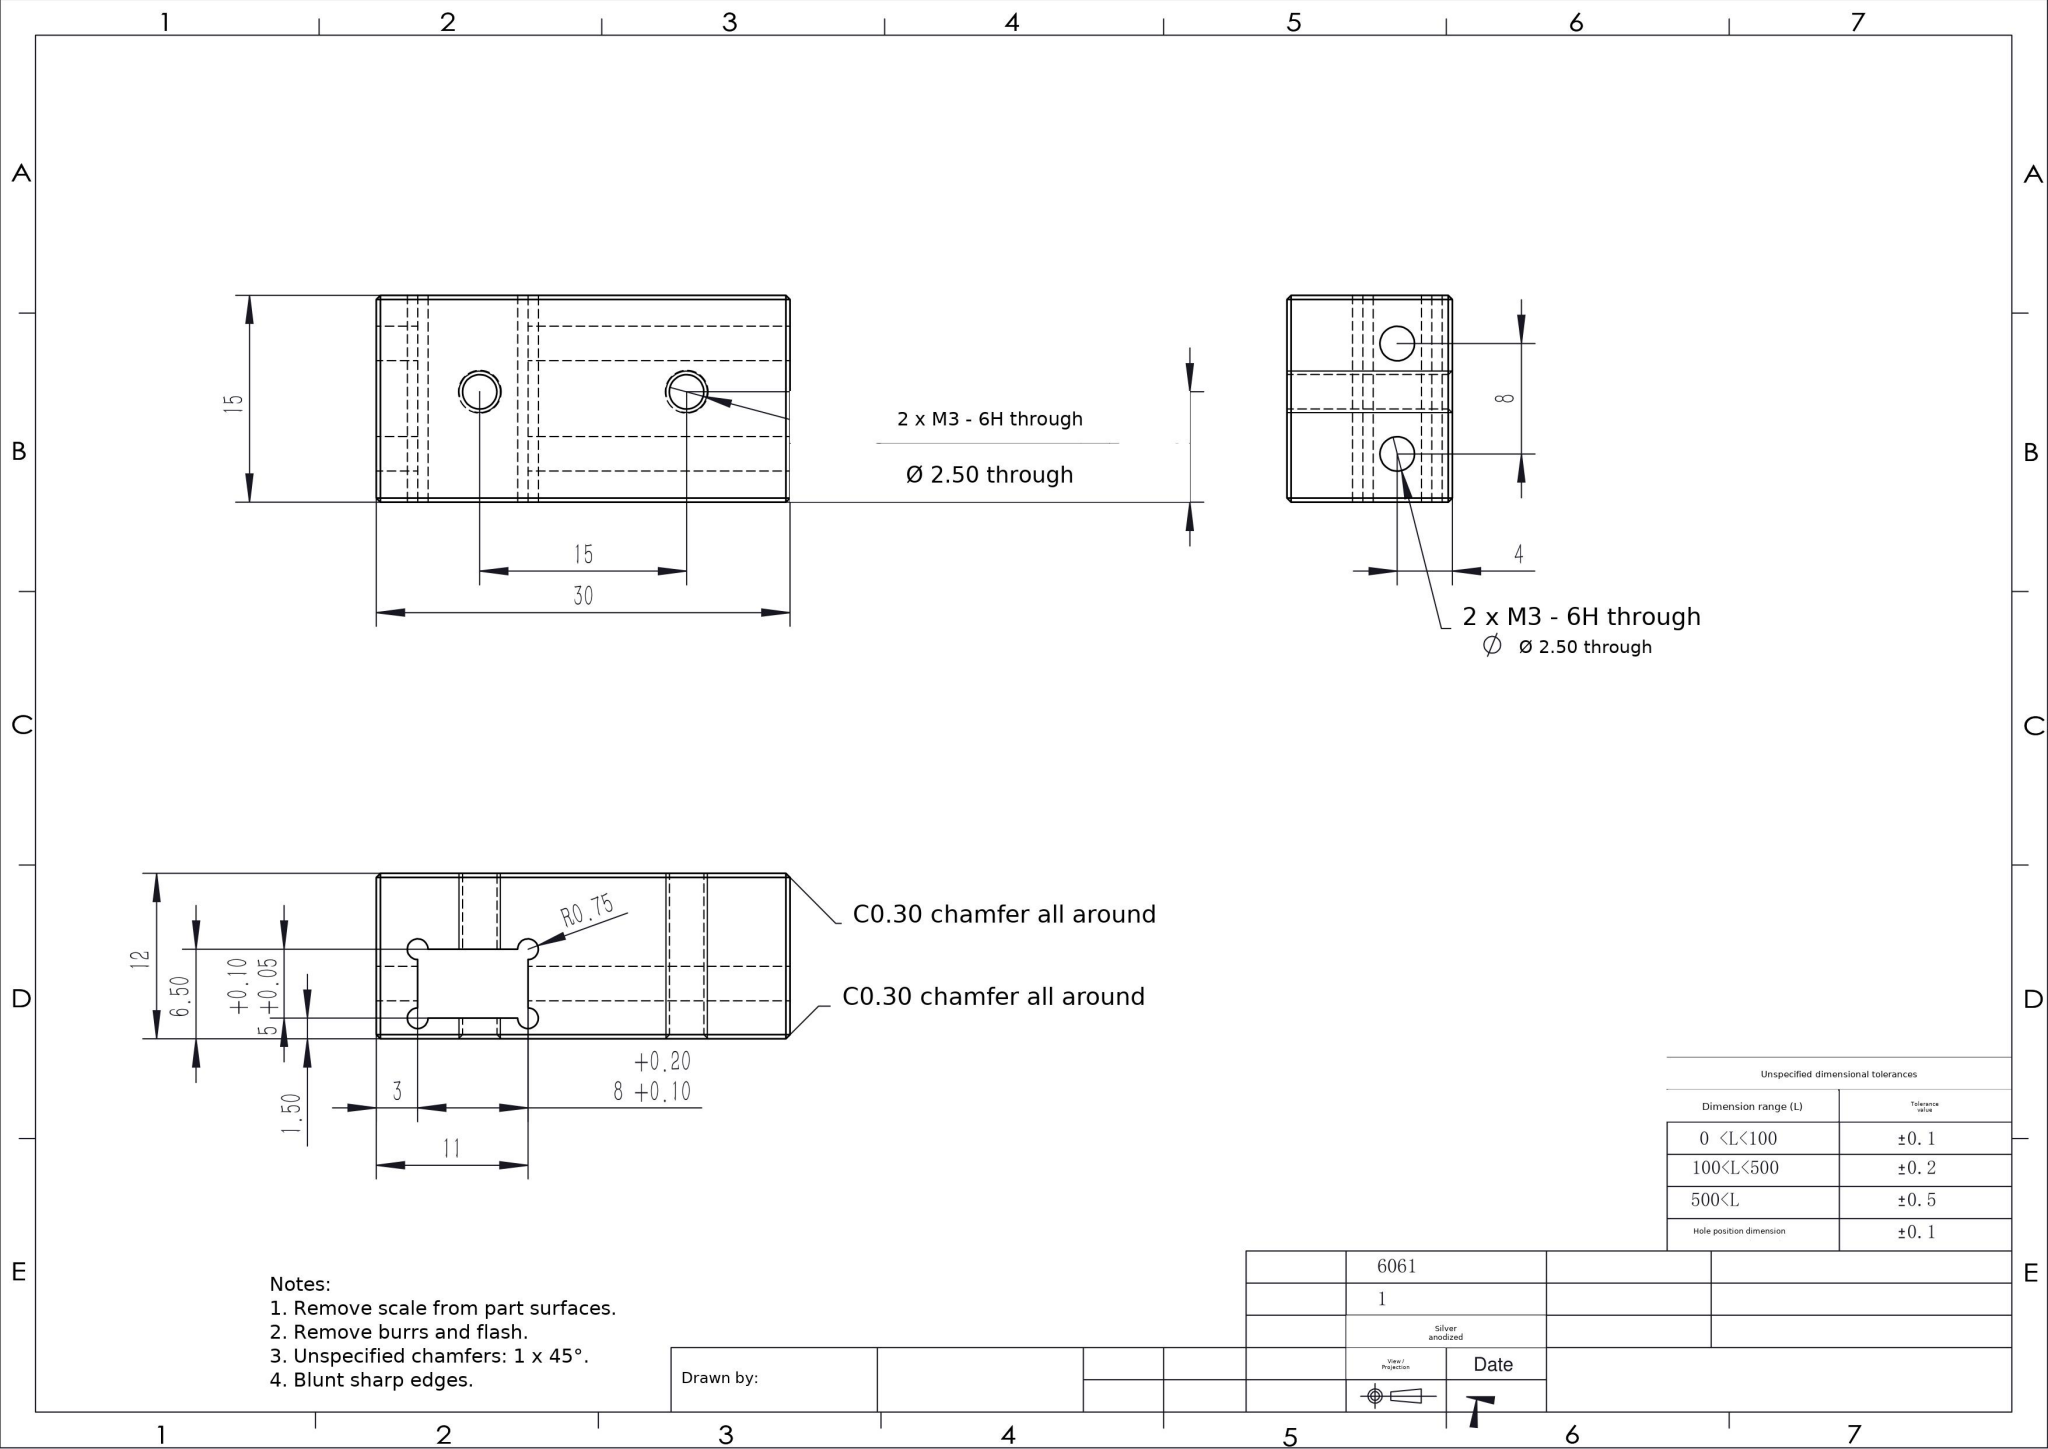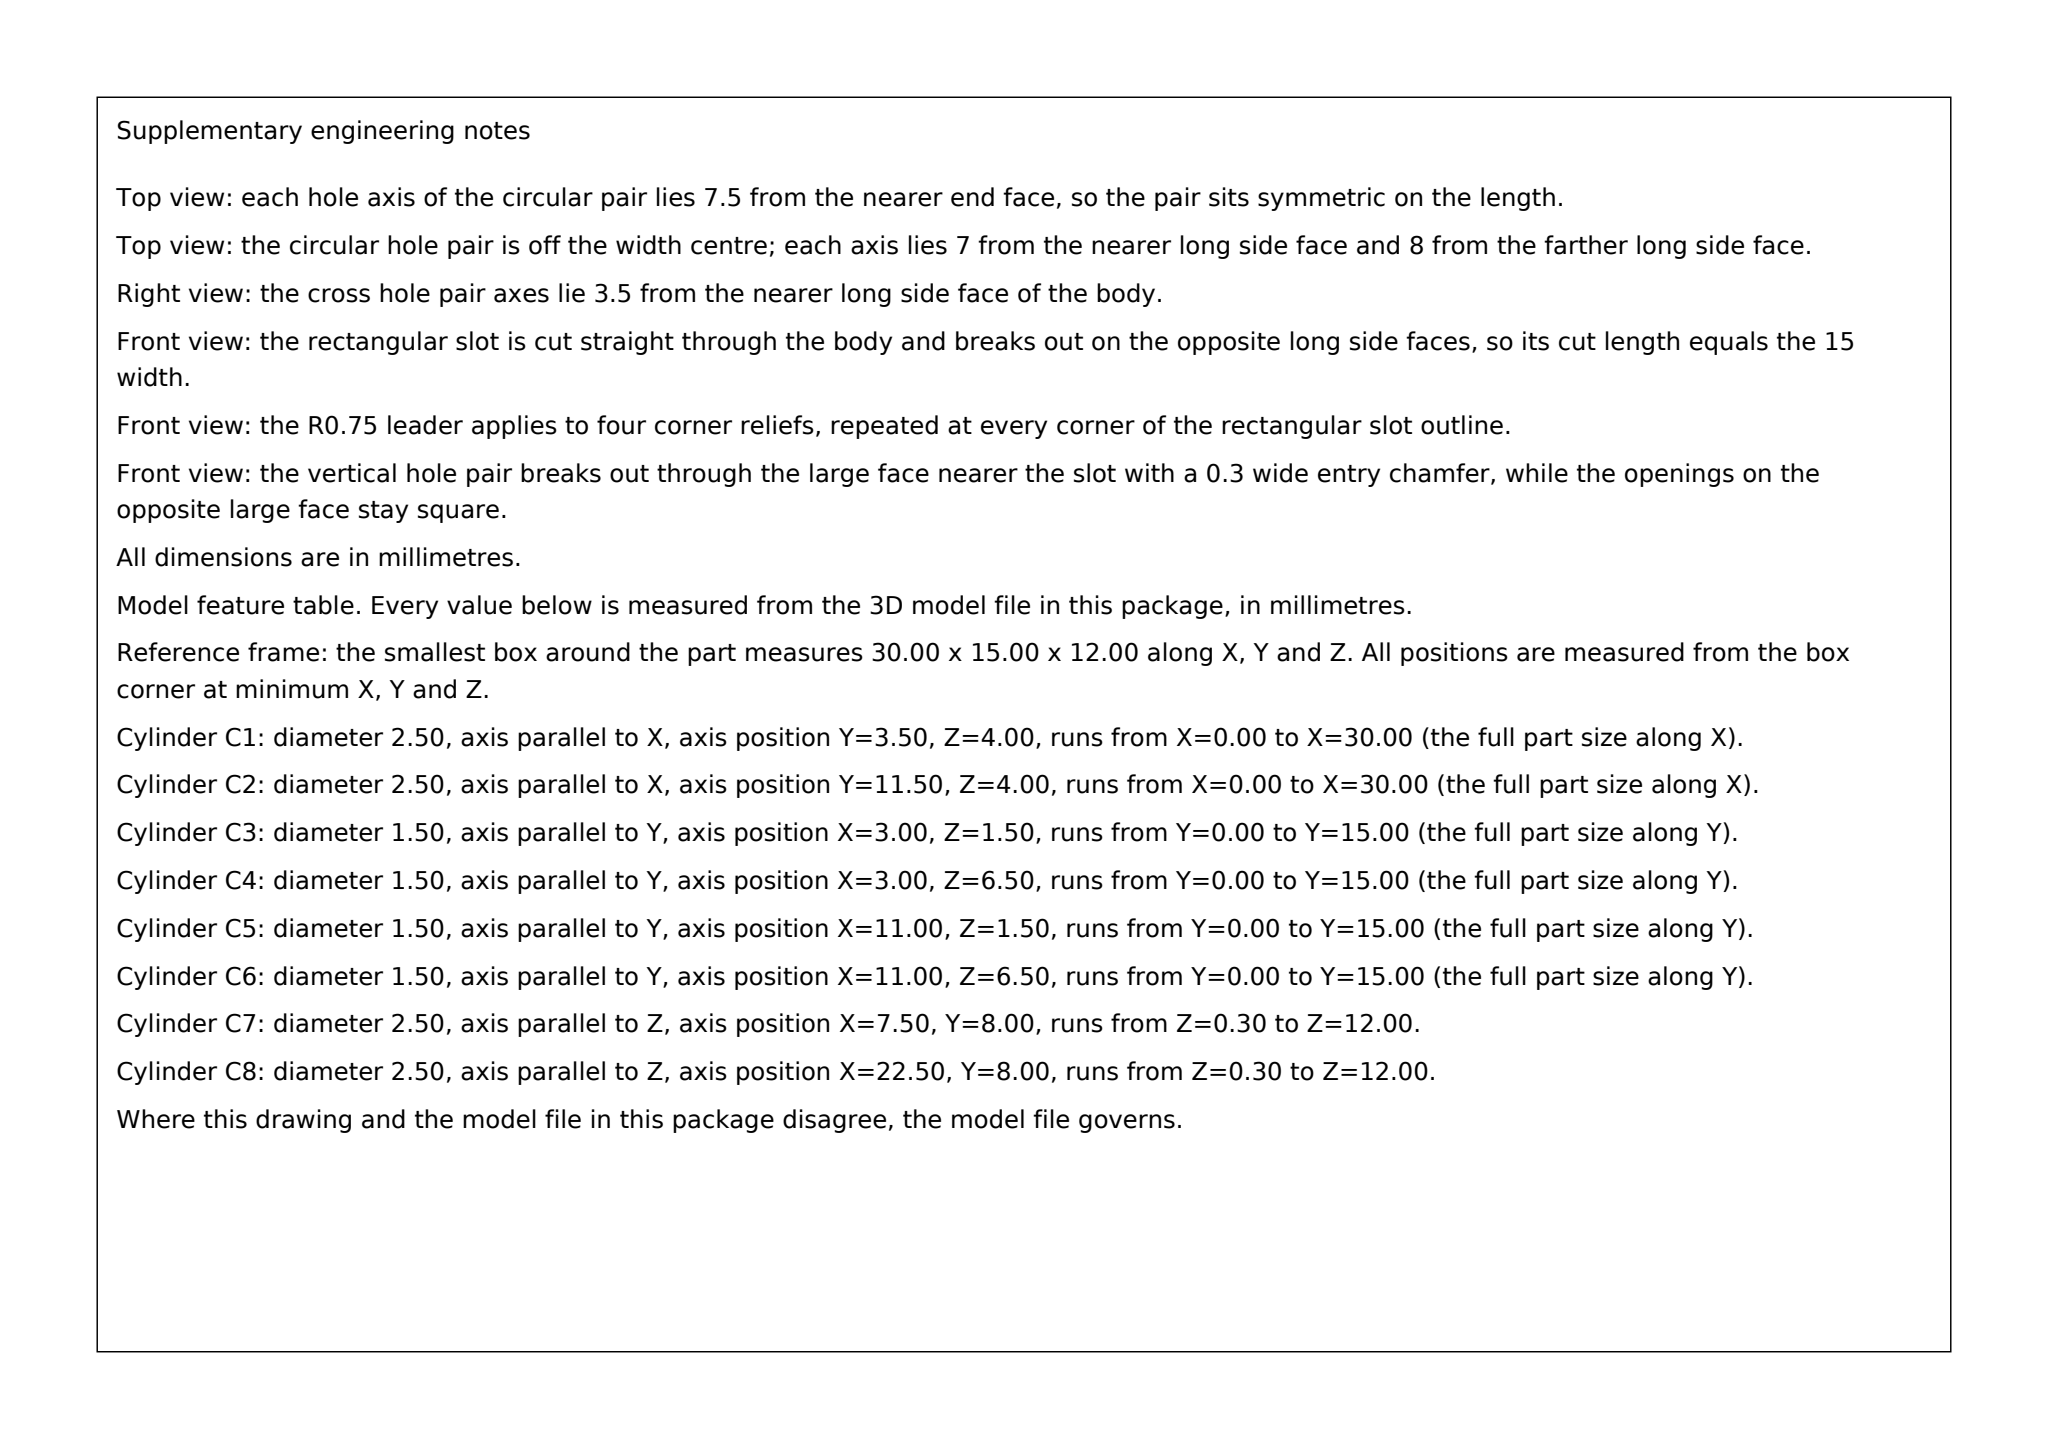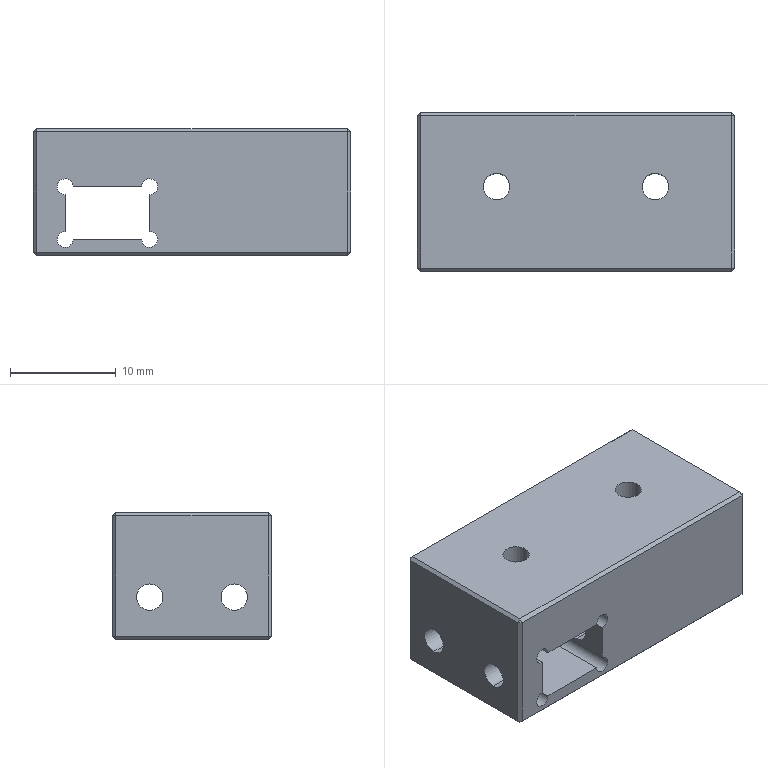Part | SolidWorks | mm | 1 solid | 54 faces | box 30 x 15 x 12 mm | volume 4400 mm3 | plane 30 | cylinder 20 | cone 4 | commonest cylinder face diameters 2.5 x14 1.5 x6
build123d program:
from build123d import *

# Parameters (mm, degrees)
SKETCH1_W           = 30
SKETCH1_H           = 15
BOSS_EXTRUDE1_DEPTH = 12
SKETCH2_W           = 8
SKETCH2_H           = 5
CUT_EXTRUDE1_DEPTH  = 25.372
M3_TAPPED_HOLE1_D   = 2.5
M3_TAPPED_HOLE2_D   = 2.5
CHAMFER1_SIZE       = 0.3
SKETCH11_R          = 0.75
CUT_EXTRUDE2_DEPTH  = 25.372


with BuildPart() as part:
    # Sketch1 → Boss-Extrude1 (new body)
    with BuildSketch(Plane.XY):
        Rectangle(SKETCH1_W, SKETCH1_H)
    extrude(amount=BOSS_EXTRUDE1_DEPTH)

    # Sketch2 → Cut-Extrude1 (cut, through all)
    with BuildSketch(Plane.XZ.offset(7.5)):
        with Locations((-8, 4)):
            Rectangle(SKETCH2_W, SKETCH2_H)
    extrude(amount=-CUT_EXTRUDE1_DEPTH, mode=Mode.SUBTRACT)

    # M3 Tapped Hole1 (through all)
    with Locations(Plane.XY.offset(12)):
        with Locations((-7.5, 0.5), (7.5, 0.5)):
            Hole(M3_TAPPED_HOLE1_D / 2)

    # M3 Tapped Hole2 (through all)
    with Locations(Plane.ZY.offset(15)):
        with Locations((4, 4), (4, -4)):
            Hole(M3_TAPPED_HOLE2_D / 2)

    # Chamfer1
    chamfer1_edges = [part.edges().sort_by_distance(p)[0] for p in [
        (-15, 0, 12),
        (0, -7.5, 12),
        (8.75, 0.5, 0),
        (-6.25, 0.5, 0),
        (15, 0, 12),
        (0, -7.5, 0),
        (-15, 0, 0),
        (0, 7.5, 0),
        (15, 0, 0),
        (0, 7.5, 12),
        (15, -7.5, 6),
        (-15, -7.5, 6),
        (-15, 7.5, 6),
        (15, 7.5, 6),
    ]]
    chamfer(chamfer1_edges, length=CHAMFER1_SIZE)

    # Sketch11 → Cut-Extrude2 (cut, through all)
    with BuildSketch(Plane(origin=(0, 7.5, 0), x_dir=(1, 0, 0), z_dir=(0, 1, 0))):
        with Locations((-4, -6.5)):
            Circle(SKETCH11_R)
        with Locations((-12, -6.5)):
            Circle(SKETCH11_R)
        with Locations((-12, -1.5)):
            Circle(SKETCH11_R)
        with Locations((-4, -1.5)):
            Circle(SKETCH11_R)
    extrude(amount=-CUT_EXTRUDE2_DEPTH, mode=Mode.SUBTRACT)


solid = part.part